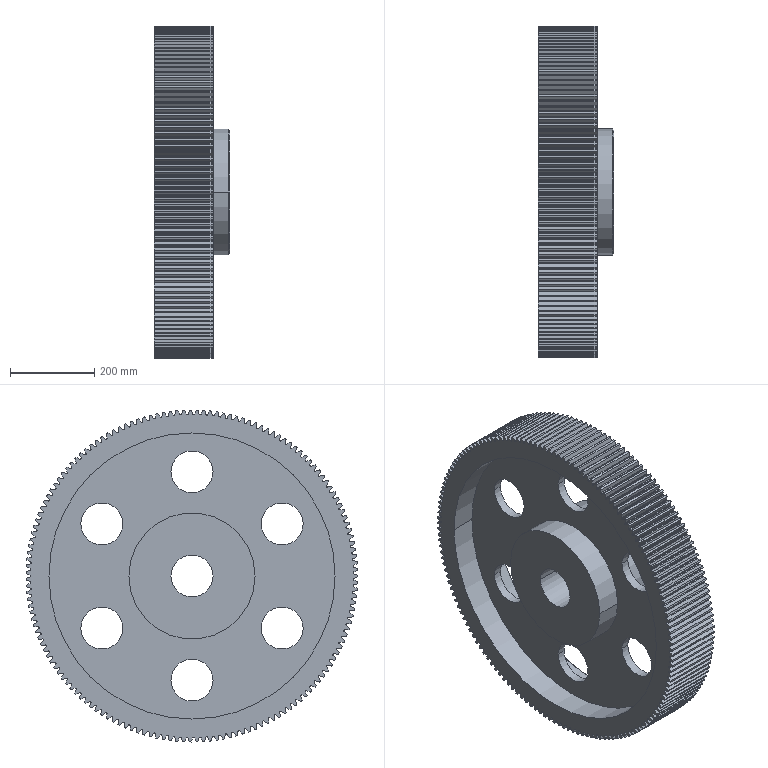Component | SolidWorks | LargeGear-1 | 1 solid | 1201 faces | volume 32125816 mm3 | cylinder 566 | plane 322 | spline 307 | cone 6 | commonest cylinder face diameters 3.8 x373 789.22 x156 100 x14 10 x12 300 x4 680 x4 270.287 x3